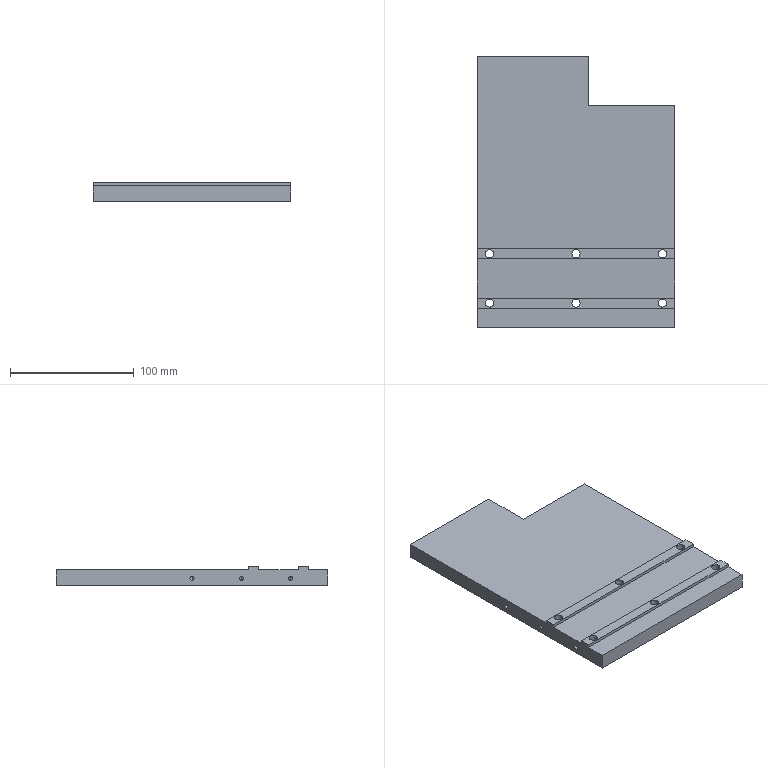Component | SolidWorks | Q1-A12-S21-Q4-11A-4 | 1 solid | 82 faces | box 160 x 220 x 15 mm | volume 405363 mm3 | cylinder 42 | plane 22 | cone 18 | commonest cylinder face diameters 3.3 x12 11 x12 6.6 x12 2.5 x6 | material White Plastic Steel POM
build123d program:
from build123d import *

# Parameters (mm, degrees)
SKETCH1_W                                            = 160
SKETCH1_H                                            = 220
BOSS_EXTRUDE1_DEPTH                                  = 15
CYLINDRICAL_COUNTERSUNK_HOLE_FOR_M6_SOCK_D           = 6.6
CYLINDRICAL_COUNTERSUNK_HOLE_FOR_M6_SOCK_CBORE_D     = 11
CYLINDRICAL_COUNTERSUNK_HOLE_FOR_M6_SOCK_CBORE_DEPTH = 6
SKETCH2_W                                            = 2.5
SKETCH2_H                                            = 15.9
SKETCH2_H_2                                          = 31.8
SKETCH2_H_3                                          = 155.9
CUT_EXTRUDE1_DEPTH                                   = 195.743
M4X0_7_TAPPED_HOLE1_D                                = 3.3
M4X0_7_TAPPED_HOLE1_DEPTH                            = 15
M4X0_7_TAPPED_HOLE1_TIP                              = 0.9914
M4X0_7_TAPPED_HOLE2_D                                = 3.3
M4X0_7_TAPPED_HOLE2_DEPTH                            = 15.5
M4X0_7_TAPPED_HOLE2_TIP                              = 0.9914
M3X0_5_TAPPED_HOLE1_D                                = 2.5
M3X0_5_TAPPED_HOLE1_DEPTH                            = 8.5
M3X0_5_TAPPED_HOLE1_TIP                              = 0.7511
SKETCH12_W                                           = 70
SKETCH12_H                                           = 40
CUT_EXTRUDE2_DEPTH                                   = 137.839


with BuildPart() as part:
    # Sketch1 → Boss-Extrude1 (new body)
    with BuildSketch(Plane.XY):
        Rectangle(SKETCH1_W, SKETCH1_H)
    extrude(amount=BOSS_EXTRUDE1_DEPTH)

    # Cylindrical Countersunk Hole for M6 Sock (through all)
    with Locations(Plane.XY.offset(15)):
        with Locations((70, -50), (70, -90), (-70, -50), (-70, -90), (0, -50), (0, -90)):
            CounterBoreHole(CYLINDRICAL_COUNTERSUNK_HOLE_FOR_M6_SOCK_D / 2, CYLINDRICAL_COUNTERSUNK_HOLE_FOR_M6_SOCK_CBORE_D / 2, CYLINDRICAL_COUNTERSUNK_HOLE_FOR_M6_SOCK_CBORE_DEPTH)

    # Sketch2 → Cut-Extrude1 (cut, through all)
    with BuildSketch(Plane(origin=(80, 0, 0), x_dir=(0, 0, -1), z_dir=(1, 0, 0))):
        with Locations((-1.25, -102.05)):
            Rectangle(SKETCH2_W, SKETCH2_H)
        with Locations((-1.25, -70)):
            Rectangle(SKETCH2_W, SKETCH2_H_2)
        with Locations((-1.25, 32.05)):
            Rectangle(SKETCH2_W, SKETCH2_H_3)
    extrude(amount=-CUT_EXTRUDE1_DEPTH, mode=Mode.SUBTRACT)

    # M4x0.7 Tapped Hole1
    with Locations(Plane(origin=(80, 0, 0), x_dir=(0, 0, -1), z_dir=(1, 0, 0))):
        with Locations((-9.5, 0), (-9.5, -40), (-9.5, -80)):
            Hole(M4X0_7_TAPPED_HOLE1_D / 2, depth=M4X0_7_TAPPED_HOLE1_DEPTH)
            with Locations((0, 0, -(M4X0_7_TAPPED_HOLE1_DEPTH + M4X0_7_TAPPED_HOLE1_TIP / 2))):  # 118° drill point
                Cone(0, M4X0_7_TAPPED_HOLE1_D / 2, M4X0_7_TAPPED_HOLE1_TIP, mode=Mode.SUBTRACT)

    # M4x0.7 Tapped Hole2
    with Locations(Plane.ZY.offset(80)):
        with Locations((9.5, 0), (9.5, -40), (9.5, -80)):
            Hole(M4X0_7_TAPPED_HOLE2_D / 2, depth=M4X0_7_TAPPED_HOLE2_DEPTH)
            with Locations((0, 0, -(M4X0_7_TAPPED_HOLE2_DEPTH + M4X0_7_TAPPED_HOLE2_TIP / 2))):  # 118° drill point
                Cone(0, M4X0_7_TAPPED_HOLE2_D / 2, M4X0_7_TAPPED_HOLE2_TIP, mode=Mode.SUBTRACT)

    # M3x0.5 Tapped Hole1
    with Locations(Plane(origin=(0, 110, 0), x_dir=(1, 0, 0), z_dir=(0, 1, 0))):
        with Locations((0, -10), (30, -10), (70, -10)):
            Hole(M3X0_5_TAPPED_HOLE1_D / 2, depth=M3X0_5_TAPPED_HOLE1_DEPTH)
            with Locations((0, 0, -(M3X0_5_TAPPED_HOLE1_DEPTH + M3X0_5_TAPPED_HOLE1_TIP / 2))):  # 118° drill point
                Cone(0, M3X0_5_TAPPED_HOLE1_D / 2, M3X0_5_TAPPED_HOLE1_TIP, mode=Mode.SUBTRACT)

    # Sketch12 → Cut-Extrude2 (cut, through all)
    with BuildSketch(Plane.XY.offset(15)):
        with Locations((-45, 90)):
            Rectangle(SKETCH12_W, SKETCH12_H)
    extrude(amount=-CUT_EXTRUDE2_DEPTH, mode=Mode.SUBTRACT)


solid = part.part

# Placed as in the assembly
solid = solid.moved(Location((298.5, 70, -147.5), (-180, 0, 180)))